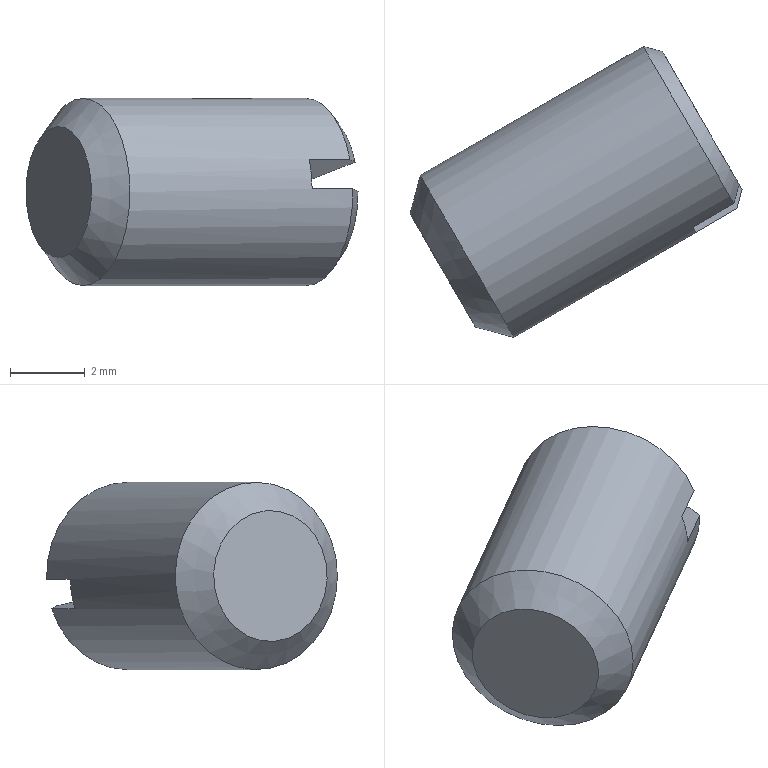Component | NX | GB-M5X8_2 | 1 solid | 10 faces | box 8.87 x 7.77 x 5 mm | volume 146 mm3 | plane 6 | cone 3 | cylinder 1 | commonest cylinder face diameters 5 x1
STEP:
#1=CARTESIAN_POINT('',(0.,0.,0.));
#2=DIRECTION('',(0.,0.,1.));
#3=DIRECTION('',(1.,0.,0.));
#4=AXIS2_PLACEMENT_3D('',#1,#2,#3);
#5=CARTESIAN_POINT('',(38.775,24.84,6.985));
#6=VERTEX_POINT('',#5);
#7=CARTESIAN_POINT('',(40.822,21.295,7.8));
#8=VERTEX_POINT('',#7);
#9=CARTESIAN_POINT('',(38.327,25.616,6.806));
#10=DIRECTION('',(0.4904,-0.8494,0.1953));
#11=VECTOR('',#10,1.);
#12=LINE('',#9,#11);
#13=CARTESIAN_POINT('',(39.837,23.,7.));
#14=DIRECTION('',(0.866,0.5,0.));
#15=DIRECTION('',(0.4904,-0.8494,0.1953));
#16=AXIS2_PLACEMENT_3D('',#13,#14,#15);
#17=PLANE('',#16);
#18=CARTESIAN_POINT('',(-3.,-0.4));
#19=DIRECTION('',(1.,0.));
#20=VECTOR('',#19,1.);
#21=LINE('',#18,#20);
#22=(GEOMETRIC_REPRESENTATION_CONTEXT(2)PARAMETRIC_REPRESENTATION_CONTEXT()REPRESENTATION_CONTEXT('',''));
#23=DEFINITIONAL_REPRESENTATION('',(#21),#22);
#24=PCURVE('',#17,#23);
#25=CARTESIAN_POINT('',(36.915,24.801,6.806));
#26=DIRECTION('',(-0.09764,0.1691,0.9807));
#27=DIRECTION('',(-0.866,-0.5,-0.));
#28=AXIS2_PLACEMENT_3D('',#25,#26,#27);
#29=PLANE('',#28);
#30=CARTESIAN_POINT('',(-1.63,0.));
#31=DIRECTION('',(0.,1.));
#32=VECTOR('',#31,1.);
#33=LINE('',#30,#32);
#34=(GEOMETRIC_REPRESENTATION_CONTEXT(2)PARAMETRIC_REPRESENTATION_CONTEXT()REPRESENTATION_CONTEXT('',''));
#35=DEFINITIONAL_REPRESENTATION('',(#33),#34);
#36=PCURVE('',#29,#35);
#37=SURFACE_CURVE('',#12,(#24,#36),.PCURVE_S1.);
#38=EDGE_CURVE('',#6,#8,#37,.T.);
#39=ORIENTED_EDGE('',*,*,#38,.F.);
#40=CARTESIAN_POINT('',(39.837,23.,7.));
#41=DIRECTION('',(0.866,0.5,-0.));
#42=DIRECTION('',(0.4904,-0.8494,0.1953));
#43=AXIS2_PLACEMENT_3D('',#40,#41,#42);
#44=CIRCLE('',#43,2.125);
#45=CARTESIAN_POINT('',(0.,0.));
#46=DIRECTION('',(1.,0.));
#47=AXIS2_PLACEMENT_2D('',#45,#46);
#48=CIRCLE('',#47,2.125);
#49=(GEOMETRIC_REPRESENTATION_CONTEXT(2)PARAMETRIC_REPRESENTATION_CONTEXT()REPRESENTATION_CONTEXT('',''));
#50=DEFINITIONAL_REPRESENTATION('',(#48),#49);
#51=PCURVE('',#17,#50);
#52=CARTESIAN_POINT('',(39.837,23.,7.));
#53=DIRECTION('',(-0.866,-0.5,0.));
#54=DIRECTION('',(-0.4904,0.8494,-0.1953));
#55=AXIS2_PLACEMENT_3D('',#52,#53,#54);
#56=CONICAL_SURFACE('',#55,2.125,0.7854);
#57=CARTESIAN_POINT('',(9.425,-0.));
#58=DIRECTION('',(-1.,0.));
#59=VECTOR('',#58,1.);
#60=LINE('',#57,#59);
#61=(GEOMETRIC_REPRESENTATION_CONTEXT(2)PARAMETRIC_REPRESENTATION_CONTEXT()REPRESENTATION_CONTEXT('',''));
#62=DEFINITIONAL_REPRESENTATION('',(#60),#61);
#63=PCURVE('',#56,#62);
#64=SURFACE_CURVE('',#44,(#51,#63),.PCURVE_S1.);
#65=EDGE_CURVE('',#6,#8,#64,.T.);
#66=ORIENTED_EDGE('',*,*,#65,.T.);
#67=EDGE_LOOP('',(#39,#66));
#68=FACE_BOUND('',#67,.T.);
#69=ADVANCED_FACE('',(#68),#17,.T.);
#70=CARTESIAN_POINT('',(38.263,24.976,6.91));
#71=VERTEX_POINT('',#70);
#72=CARTESIAN_POINT('',(38.263,24.976,6.91));
#73=CARTESIAN_POINT('',(38.434,24.931,6.935));
#74=CARTESIAN_POINT('',(38.604,24.886,6.96));
#75=CARTESIAN_POINT('',(38.775,24.84,6.985));
#76=B_SPLINE_CURVE_WITH_KNOTS('',3,(#72,#73,#74,#75),.UNSPECIFIED.,.F.,.F.,(4,4),(0.,1.),.PIECEWISE_BEZIER_KNOTS.);
#77=CARTESIAN_POINT('',(6.122,0.375));
#78=CARTESIAN_POINT('',(6.094,-0.));
#79=B_SPLINE_CURVE_WITH_KNOTS('',1,(#77,#78),.UNSPECIFIED.,.F.,.F.,(2,2),(0.,1.),.PIECEWISE_BEZIER_KNOTS.);
#80=(GEOMETRIC_REPRESENTATION_CONTEXT(2)PARAMETRIC_REPRESENTATION_CONTEXT()REPRESENTATION_CONTEXT('',''));
#81=DEFINITIONAL_REPRESENTATION('',(#79),#80);
#82=PCURVE('',#56,#81);
#83=CARTESIAN_POINT('',(-1.255,0.5322));
#84=CARTESIAN_POINT('',(-1.38,0.659));
#85=CARTESIAN_POINT('',(-1.505,0.7859));
#86=CARTESIAN_POINT('',(-1.63,0.913));
#87=B_SPLINE_CURVE_WITH_KNOTS('',3,(#83,#84,#85,#86),.UNSPECIFIED.,.F.,.F.,(4,4),(0.,1.),.PIECEWISE_BEZIER_KNOTS.);
#88=(GEOMETRIC_REPRESENTATION_CONTEXT(2)PARAMETRIC_REPRESENTATION_CONTEXT()REPRESENTATION_CONTEXT('',''));
#89=DEFINITIONAL_REPRESENTATION('',(#87),#88);
#90=PCURVE('',#29,#89);
#91=SURFACE_CURVE('',#76,(#82,#90),.PCURVE_S1.);
#92=EDGE_CURVE('',#71,#6,#91,.T.);
#93=ORIENTED_EDGE('',*,*,#92,.F.);
#94=CARTESIAN_POINT('',(40.683,20.784,7.874));
#95=VERTEX_POINT('',#94);
#96=CARTESIAN_POINT('',(39.512,22.812,7.));
#97=DIRECTION('',(-0.866,-0.5,0.));
#98=DIRECTION('',(0.4904,-0.8494,0.1953));
#99=AXIS2_PLACEMENT_3D('',#96,#97,#98);
#100=CIRCLE('',#99,2.5);
#101=CARTESIAN_POINT('',(3.142,0.375));
#102=DIRECTION('',(1.,-0.));
#103=VECTOR('',#102,1.);
#104=LINE('',#101,#103);
#105=(GEOMETRIC_REPRESENTATION_CONTEXT(2)PARAMETRIC_REPRESENTATION_CONTEXT()REPRESENTATION_CONTEXT('',''));
#106=DEFINITIONAL_REPRESENTATION('',(#104),#105);
#107=PCURVE('',#56,#106);
#108=CARTESIAN_POINT('',(39.837,23.,7.));
#109=DIRECTION('',(-0.866,-0.5,0.));
#110=DIRECTION('',(-0.4904,0.8494,-0.1953));
#111=AXIS2_PLACEMENT_3D('',#108,#109,#110);
#112=CYLINDRICAL_SURFACE('',#111,2.5);
#113=CARTESIAN_POINT('',(3.142,0.375));
#114=DIRECTION('',(1.,0.));
#115=VECTOR('',#114,1.);
#116=LINE('',#113,#115);
#117=(GEOMETRIC_REPRESENTATION_CONTEXT(2)PARAMETRIC_REPRESENTATION_CONTEXT()REPRESENTATION_CONTEXT('',''));
#118=DEFINITIONAL_REPRESENTATION('',(#116),#117);
#119=PCURVE('',#112,#118);
#120=SURFACE_CURVE('',#100,(#107,#119),.PCURVE_S1.);
#121=EDGE_CURVE('',#95,#71,#120,.T.);
#122=ORIENTED_EDGE('',*,*,#121,.F.);
#123=CARTESIAN_POINT('',(40.822,21.295,7.8));
#124=CARTESIAN_POINT('',(40.781,21.144,7.822));
#125=CARTESIAN_POINT('',(40.74,20.994,7.844));
#126=CARTESIAN_POINT('',(40.7,20.843,7.866));
#127=CARTESIAN_POINT('',(40.694,20.824,7.868));
#128=CARTESIAN_POINT('',(40.689,20.804,7.871));
#129=CARTESIAN_POINT('',(40.683,20.784,7.874));
#130=B_SPLINE_CURVE_WITH_KNOTS('',3,(#123,#124,#125,#126,#127,#128,#129),.UNSPECIFIED.,.F.,.F.,(4,3,4),(0.,0.8839,1.),.UNSPECIFIED.);
#131=CARTESIAN_POINT('',(3.331,-0.));
#132=CARTESIAN_POINT('',(3.302,0.375));
#133=B_SPLINE_CURVE_WITH_KNOTS('',1,(#131,#132),.UNSPECIFIED.,.F.,.F.,(2,2),(0.,1.),.PIECEWISE_BEZIER_KNOTS.);
#134=(GEOMETRIC_REPRESENTATION_CONTEXT(2)PARAMETRIC_REPRESENTATION_CONTEXT()REPRESENTATION_CONTEXT('',''));
#135=DEFINITIONAL_REPRESENTATION('',(#133),#134);
#136=PCURVE('',#56,#135);
#137=CARTESIAN_POINT('',(-1.63,5.087));
#138=CARTESIAN_POINT('',(-1.52,5.199));
#139=CARTESIAN_POINT('',(-1.409,5.312));
#140=CARTESIAN_POINT('',(-1.299,5.424));
#141=CARTESIAN_POINT('',(-1.284,5.438));
#142=CARTESIAN_POINT('',(-1.27,5.453));
#143=CARTESIAN_POINT('',(-1.255,5.468));
#144=B_SPLINE_CURVE_WITH_KNOTS('',3,(#137,#138,#139,#140,#141,#142,#143),.UNSPECIFIED.,.F.,.F.,(4,3,4),(0.,0.8839,1.),.UNSPECIFIED.);
#145=(GEOMETRIC_REPRESENTATION_CONTEXT(2)PARAMETRIC_REPRESENTATION_CONTEXT()REPRESENTATION_CONTEXT('',''));
#146=DEFINITIONAL_REPRESENTATION('',(#144),#145);
#147=PCURVE('',#29,#146);
#148=SURFACE_CURVE('',#130,(#136,#147),.PCURVE_S1.);
#149=EDGE_CURVE('',#8,#95,#148,.T.);
#150=ORIENTED_EDGE('',*,*,#149,.F.);
#151=ORIENTED_EDGE('',*,*,#65,.F.);
#152=EDGE_LOOP('',(#93,#122,#150,#151));
#153=FACE_BOUND('',#152,.T.);
#154=ADVANCED_FACE('',(#153),#56,.T.);
#155=ORIENTED_EDGE('',*,*,#121,.T.);
#156=CARTESIAN_POINT('',(37.176,24.349,6.91));
#157=VERTEX_POINT('',#156);
#158=CARTESIAN_POINT('',(38.588,25.164,6.91));
#159=DIRECTION('',(-0.866,-0.5,0.));
#160=VECTOR('',#159,1.);
#161=LINE('',#158,#160);
#162=CARTESIAN_POINT('',(6.122,-0.));
#163=DIRECTION('',(0.,1.));
#164=VECTOR('',#163,1.);
#165=LINE('',#162,#164);
#166=(GEOMETRIC_REPRESENTATION_CONTEXT(2)PARAMETRIC_REPRESENTATION_CONTEXT()REPRESENTATION_CONTEXT('',''));
#167=DEFINITIONAL_REPRESENTATION('',(#165),#166);
#168=PCURVE('',#112,#167);
#169=CARTESIAN_POINT('',(-1.63,0.5322));
#170=DIRECTION('',(1.,-0.));
#171=VECTOR('',#170,1.);
#172=LINE('',#169,#171);
#173=(GEOMETRIC_REPRESENTATION_CONTEXT(2)PARAMETRIC_REPRESENTATION_CONTEXT()REPRESENTATION_CONTEXT('',''));
#174=DEFINITIONAL_REPRESENTATION('',(#172),#173);
#175=PCURVE('',#29,#174);
#176=SURFACE_CURVE('',#161,(#168,#175),.PCURVE_S1.);
#177=EDGE_CURVE('',#71,#157,#176,.T.);
#178=ORIENTED_EDGE('',*,*,#177,.T.);
#179=CARTESIAN_POINT('',(37.254,24.213,6.126));
#180=VERTEX_POINT('',#179);
#181=CARTESIAN_POINT('',(38.426,22.185,7.));
#182=DIRECTION('',(0.866,0.5,0.));
#183=DIRECTION('',(0.4904,-0.8494,0.1953));
#184=AXIS2_PLACEMENT_3D('',#181,#182,#183);
#185=CIRCLE('',#184,2.5);
#186=CARTESIAN_POINT('',(9.425,1.63));
#187=DIRECTION('',(-1.,0.));
#188=VECTOR('',#187,1.);
#189=LINE('',#186,#188);
#190=(GEOMETRIC_REPRESENTATION_CONTEXT(2)PARAMETRIC_REPRESENTATION_CONTEXT()REPRESENTATION_CONTEXT('',''));
#191=DEFINITIONAL_REPRESENTATION('',(#189),#190);
#192=PCURVE('',#112,#191);
#193=CARTESIAN_POINT('',(38.426,22.185,7.));
#194=DIRECTION('',(0.866,0.5,0.));
#195=DIRECTION('',(0.4904,-0.8494,0.1953));
#196=AXIS2_PLACEMENT_3D('',#193,#194,#195);
#197=PLANE('',#196);
#198=CARTESIAN_POINT('',(0.,0.));
#199=DIRECTION('',(1.,-0.));
#200=AXIS2_PLACEMENT_2D('',#198,#199);
#201=CIRCLE('',#200,2.5);
#202=(GEOMETRIC_REPRESENTATION_CONTEXT(2)PARAMETRIC_REPRESENTATION_CONTEXT()REPRESENTATION_CONTEXT('',''));
#203=DEFINITIONAL_REPRESENTATION('',(#201),#202);
#204=PCURVE('',#197,#203);
#205=SURFACE_CURVE('',#185,(#192,#204),.PCURVE_S1.);
#206=EDGE_CURVE('',#180,#157,#205,.T.);
#207=ORIENTED_EDGE('',*,*,#206,.F.);
#208=CARTESIAN_POINT('',(32.387,21.403,6.126));
#209=VERTEX_POINT('',#208);
#210=CARTESIAN_POINT('',(37.254,24.213,6.126));
#211=CARTESIAN_POINT('',(32.387,21.403,6.126));
#212=B_SPLINE_CURVE_WITH_KNOTS('',1,(#210,#211),.UNSPECIFIED.,.F.,.F.,(2,2),(1.63,7.25),.PIECEWISE_BEZIER_KNOTS.);
#213=CARTESIAN_POINT('',(6.444,0.));
#214=DIRECTION('',(0.,1.));
#215=VECTOR('',#214,1.);
#216=LINE('',#213,#215);
#217=(GEOMETRIC_REPRESENTATION_CONTEXT(2)PARAMETRIC_REPRESENTATION_CONTEXT()REPRESENTATION_CONTEXT('',''));
#218=DEFINITIONAL_REPRESENTATION('',(#216),#217);
#219=PCURVE('',#112,#218);
#220=CARTESIAN_POINT('',(0.1607,0.));
#221=DIRECTION('',(0.,1.));
#222=VECTOR('',#221,1.);
#223=LINE('',#220,#222);
#224=(GEOMETRIC_REPRESENTATION_CONTEXT(2)PARAMETRIC_REPRESENTATION_CONTEXT()REPRESENTATION_CONTEXT('',''));
#225=DEFINITIONAL_REPRESENTATION('',(#223),#224);
#226=PCURVE('',#112,#225);
#227=SEAM_CURVE('',#212,(#219,#226),.PCURVE_S1.);
#228=EDGE_CURVE('',#180,#209,#227,.T.);
#229=ORIENTED_EDGE('',*,*,#228,.T.);
#230=CARTESIAN_POINT('',(34.784,17.252,7.488));
#231=VERTEX_POINT('',#230);
#232=CARTESIAN_POINT('',(33.558,19.375,7.));
#233=DIRECTION('',(0.866,0.5,0.));
#234=DIRECTION('',(0.4904,-0.8494,0.1953));
#235=AXIS2_PLACEMENT_3D('',#232,#233,#234);
#236=CIRCLE('',#235,2.5);
#237=CARTESIAN_POINT('',(9.425,7.25));
#238=DIRECTION('',(-1.,0.));
#239=VECTOR('',#238,1.);
#240=LINE('',#237,#239);
#241=(GEOMETRIC_REPRESENTATION_CONTEXT(2)PARAMETRIC_REPRESENTATION_CONTEXT()REPRESENTATION_CONTEXT('',''));
#242=DEFINITIONAL_REPRESENTATION('',(#240),#241);
#243=PCURVE('',#112,#242);
#244=CARTESIAN_POINT('',(33.558,19.375,7.));
#245=DIRECTION('',(0.866,0.5,0.));
#246=DIRECTION('',(0.4904,-0.8494,0.1953));
#247=AXIS2_PLACEMENT_3D('',#244,#245,#246);
#248=CONICAL_SURFACE('',#247,2.5,0.7854);
#249=CARTESIAN_POINT('',(0.,0.));
#250=DIRECTION('',(1.,-0.));
#251=VECTOR('',#250,1.);
#252=LINE('',#249,#251);
#253=(GEOMETRIC_REPRESENTATION_CONTEXT(2)PARAMETRIC_REPRESENTATION_CONTEXT()REPRESENTATION_CONTEXT('',''));
#254=DEFINITIONAL_REPRESENTATION('',(#252),#253);
#255=PCURVE('',#248,#254);
#256=SURFACE_CURVE('',#236,(#243,#255),.PCURVE_S1.);
#257=EDGE_CURVE('',#209,#231,#256,.T.);
#258=ORIENTED_EDGE('',*,*,#257,.T.);
#259=CARTESIAN_POINT('',(33.558,19.375,7.));
#260=DIRECTION('',(0.866,0.5,0.));
#261=DIRECTION('',(0.4904,-0.8494,0.1953));
#262=AXIS2_PLACEMENT_3D('',#259,#260,#261);
#263=CIRCLE('',#262,2.5);
#264=CARTESIAN_POINT('',(3.142,7.25));
#265=DIRECTION('',(-1.,0.));
#266=VECTOR('',#265,1.);
#267=LINE('',#264,#266);
#268=(GEOMETRIC_REPRESENTATION_CONTEXT(2)PARAMETRIC_REPRESENTATION_CONTEXT()REPRESENTATION_CONTEXT('',''));
#269=DEFINITIONAL_REPRESENTATION('',(#267),#268);
#270=PCURVE('',#112,#269);
#271=CARTESIAN_POINT('',(0.,-0.));
#272=DIRECTION('',(1.,0.));
#273=VECTOR('',#272,1.);
#274=LINE('',#271,#273);
#275=(GEOMETRIC_REPRESENTATION_CONTEXT(2)PARAMETRIC_REPRESENTATION_CONTEXT()REPRESENTATION_CONTEXT('',''));
#276=DEFINITIONAL_REPRESENTATION('',(#274),#275);
#277=PCURVE('',#248,#276);
#278=SURFACE_CURVE('',#263,(#270,#277),.PCURVE_S1.);
#279=EDGE_CURVE('',#231,#209,#278,.T.);
#280=ORIENTED_EDGE('',*,*,#279,.T.);
#281=ORIENTED_EDGE('',*,*,#228,.F.);
#282=CARTESIAN_POINT('',(38.341,24.841,6.126));
#283=VERTEX_POINT('',#282);
#284=CARTESIAN_POINT('',(38.666,25.028,6.126));
#285=DIRECTION('',(0.866,0.5,0.));
#286=VECTOR('',#285,1.);
#287=LINE('',#284,#286);
#288=CARTESIAN_POINT('',(0.1607,-0.));
#289=DIRECTION('',(0.,-1.));
#290=VECTOR('',#289,1.);
#291=LINE('',#288,#290);
#292=(GEOMETRIC_REPRESENTATION_CONTEXT(2)PARAMETRIC_REPRESENTATION_CONTEXT()REPRESENTATION_CONTEXT('',''));
#293=DEFINITIONAL_REPRESENTATION('',(#291),#292);
#294=PCURVE('',#112,#293);
#295=CARTESIAN_POINT('',(39.936,19.569,7.194));
#296=DIRECTION('',(0.09764,-0.1691,-0.9807));
#297=DIRECTION('',(0.866,0.5,0.));
#298=AXIS2_PLACEMENT_3D('',#295,#296,#297);
#299=PLANE('',#298);
#300=CARTESIAN_POINT('',(1.63,-5.468));
#301=DIRECTION('',(1.,0.));
#302=VECTOR('',#301,1.);
#303=LINE('',#300,#302);
#304=(GEOMETRIC_REPRESENTATION_CONTEXT(2)PARAMETRIC_REPRESENTATION_CONTEXT()REPRESENTATION_CONTEXT('',''));
#305=DEFINITIONAL_REPRESENTATION('',(#303),#304);
#306=PCURVE('',#299,#305);
#307=SURFACE_CURVE('',#287,(#294,#306),.PCURVE_S1.);
#308=EDGE_CURVE('',#180,#283,#307,.T.);
#309=ORIENTED_EDGE('',*,*,#308,.T.);
#310=CARTESIAN_POINT('',(40.762,20.649,7.09));
#311=VERTEX_POINT('',#310);
#312=CARTESIAN_POINT('',(39.512,22.812,7.));
#313=DIRECTION('',(-0.866,-0.5,0.));
#314=DIRECTION('',(0.4904,-0.8494,0.1953));
#315=AXIS2_PLACEMENT_3D('',#312,#313,#314);
#316=CIRCLE('',#315,2.5);
#317=CARTESIAN_POINT('',(-3.142,0.375));
#318=DIRECTION('',(1.,0.));
#319=VECTOR('',#318,1.);
#320=LINE('',#317,#319);
#321=(GEOMETRIC_REPRESENTATION_CONTEXT(2)PARAMETRIC_REPRESENTATION_CONTEXT()REPRESENTATION_CONTEXT('',''));
#322=DEFINITIONAL_REPRESENTATION('',(#320),#321);
#323=PCURVE('',#112,#322);
#324=CARTESIAN_POINT('',(39.837,23.,7.));
#325=DIRECTION('',(-0.866,-0.5,0.));
#326=DIRECTION('',(-0.4904,0.8494,-0.1953));
#327=AXIS2_PLACEMENT_3D('',#324,#325,#326);
#328=CONICAL_SURFACE('',#327,2.125,0.7854);
#329=CARTESIAN_POINT('',(-3.142,0.375));
#330=DIRECTION('',(1.,0.));
#331=VECTOR('',#330,1.);
#332=LINE('',#329,#331);
#333=(GEOMETRIC_REPRESENTATION_CONTEXT(2)PARAMETRIC_REPRESENTATION_CONTEXT()REPRESENTATION_CONTEXT('',''));
#334=DEFINITIONAL_REPRESENTATION('',(#332),#333);
#335=PCURVE('',#328,#334);
#336=SURFACE_CURVE('',#316,(#323,#335),.PCURVE_S1.);
#337=EDGE_CURVE('',#283,#311,#336,.T.);
#338=ORIENTED_EDGE('',*,*,#337,.T.);
#339=CARTESIAN_POINT('',(39.675,20.021,7.09));
#340=VERTEX_POINT('',#339);
#341=CARTESIAN_POINT('',(41.086,20.836,7.09));
#342=DIRECTION('',(-0.866,-0.5,0.));
#343=VECTOR('',#342,1.);
#344=LINE('',#341,#343);
#345=CARTESIAN_POINT('',(2.981,-0.));
#346=DIRECTION('',(0.,1.));
#347=VECTOR('',#346,1.);
#348=LINE('',#345,#347);
#349=(GEOMETRIC_REPRESENTATION_CONTEXT(2)PARAMETRIC_REPRESENTATION_CONTEXT()REPRESENTATION_CONTEXT('',''));
#350=DEFINITIONAL_REPRESENTATION('',(#348),#349);
#351=PCURVE('',#112,#350);
#352=CARTESIAN_POINT('',(1.63,-0.5322));
#353=DIRECTION('',(-1.,-0.));
#354=VECTOR('',#353,1.);
#355=LINE('',#352,#354);
#356=(GEOMETRIC_REPRESENTATION_CONTEXT(2)PARAMETRIC_REPRESENTATION_CONTEXT()REPRESENTATION_CONTEXT('',''));
#357=DEFINITIONAL_REPRESENTATION('',(#355),#356);
#358=PCURVE('',#299,#357);
#359=SURFACE_CURVE('',#344,(#351,#358),.PCURVE_S1.);
#360=EDGE_CURVE('',#311,#340,#359,.T.);
#361=ORIENTED_EDGE('',*,*,#360,.T.);
#362=CARTESIAN_POINT('',(39.597,20.157,7.874));
#363=VERTEX_POINT('',#362);
#364=CARTESIAN_POINT('',(38.426,22.185,7.));
#365=DIRECTION('',(0.866,0.5,0.));
#366=DIRECTION('',(0.4904,-0.8494,0.1953));
#367=AXIS2_PLACEMENT_3D('',#364,#365,#366);
#368=CIRCLE('',#367,2.5);
#369=CARTESIAN_POINT('',(9.425,1.63));
#370=DIRECTION('',(-1.,0.));
#371=VECTOR('',#370,1.);
#372=LINE('',#369,#371);
#373=(GEOMETRIC_REPRESENTATION_CONTEXT(2)PARAMETRIC_REPRESENTATION_CONTEXT()REPRESENTATION_CONTEXT('',''));
#374=DEFINITIONAL_REPRESENTATION('',(#372),#373);
#375=PCURVE('',#112,#374);
#376=CARTESIAN_POINT('',(0.,0.));
#377=DIRECTION('',(1.,-0.));
#378=AXIS2_PLACEMENT_2D('',#376,#377);
#379=CIRCLE('',#378,2.5);
#380=(GEOMETRIC_REPRESENTATION_CONTEXT(2)PARAMETRIC_REPRESENTATION_CONTEXT()REPRESENTATION_CONTEXT('',''));
#381=DEFINITIONAL_REPRESENTATION('',(#379),#380);
#382=PCURVE('',#197,#381);
#383=SURFACE_CURVE('',#368,(#375,#382),.PCURVE_S1.);
#384=EDGE_CURVE('',#363,#340,#383,.T.);
#385=ORIENTED_EDGE('',*,*,#384,.F.);
#386=CARTESIAN_POINT('',(41.008,20.972,7.874));
#387=DIRECTION('',(0.866,0.5,0.));
#388=VECTOR('',#387,1.);
#389=LINE('',#386,#388);
#390=CARTESIAN_POINT('',(3.302,-0.));
#391=DIRECTION('',(0.,-1.));
#392=VECTOR('',#391,1.);
#393=LINE('',#390,#392);
#394=(GEOMETRIC_REPRESENTATION_CONTEXT(2)PARAMETRIC_REPRESENTATION_CONTEXT()REPRESENTATION_CONTEXT('',''));
#395=DEFINITIONAL_REPRESENTATION('',(#393),#394);
#396=PCURVE('',#112,#395);
#397=CARTESIAN_POINT('',(-1.63,5.468));
#398=DIRECTION('',(-1.,0.));
#399=VECTOR('',#398,1.);
#400=LINE('',#397,#399);
#401=(GEOMETRIC_REPRESENTATION_CONTEXT(2)PARAMETRIC_REPRESENTATION_CONTEXT()REPRESENTATION_CONTEXT('',''));
#402=DEFINITIONAL_REPRESENTATION('',(#400),#401);
#403=PCURVE('',#29,#402);
#404=SURFACE_CURVE('',#389,(#396,#403),.PCURVE_S1.);
#405=EDGE_CURVE('',#363,#95,#404,.T.);
#406=ORIENTED_EDGE('',*,*,#405,.T.);
#407=EDGE_LOOP('',(#155,#178,#207,#229,#258,#280,#281,#309,#338,#361,#385,#406));
#408=FACE_BOUND('',#407,.T.);
#409=ADVANCED_FACE('',(#408),#112,.T.);
#410=CARTESIAN_POINT('',(40.9,21.16,7.015));
#411=VERTEX_POINT('',#410);
#412=CARTESIAN_POINT('',(38.853,24.705,6.2));
#413=VERTEX_POINT('',#412);
#414=CARTESIAN_POINT('',(41.347,20.384,7.194));
#415=DIRECTION('',(-0.4904,0.8494,-0.1953));
#416=VECTOR('',#415,1.);
#417=LINE('',#414,#416);
#418=CARTESIAN_POINT('',(39.837,23.,7.));
#419=DIRECTION('',(0.866,0.5,0.));
#420=DIRECTION('',(0.4904,-0.8494,0.1953));
#421=AXIS2_PLACEMENT_3D('',#418,#419,#420);
#422=PLANE('',#421);
#423=CARTESIAN_POINT('',(3.,0.4));
#424=DIRECTION('',(-1.,0.));
#425=VECTOR('',#424,1.);
#426=LINE('',#423,#425);
#427=(GEOMETRIC_REPRESENTATION_CONTEXT(2)PARAMETRIC_REPRESENTATION_CONTEXT()REPRESENTATION_CONTEXT('',''));
#428=DEFINITIONAL_REPRESENTATION('',(#426),#427);
#429=PCURVE('',#422,#428);
#430=CARTESIAN_POINT('',(1.63,-0.));
#431=DIRECTION('',(0.,-1.));
#432=VECTOR('',#431,1.);
#433=LINE('',#430,#432);
#434=(GEOMETRIC_REPRESENTATION_CONTEXT(2)PARAMETRIC_REPRESENTATION_CONTEXT()REPRESENTATION_CONTEXT('',''));
#435=DEFINITIONAL_REPRESENTATION('',(#433),#434);
#436=PCURVE('',#299,#435);
#437=SURFACE_CURVE('',#417,(#429,#436),.PCURVE_S1.);
#438=EDGE_CURVE('',#411,#413,#437,.T.);
#439=ORIENTED_EDGE('',*,*,#438,.F.);
#440=CARTESIAN_POINT('',(39.837,23.,7.));
#441=DIRECTION('',(0.866,0.5,-0.));
#442=DIRECTION('',(0.4904,-0.8494,0.1953));
#443=AXIS2_PLACEMENT_3D('',#440,#441,#442);
#444=CIRCLE('',#443,2.125);
#445=CARTESIAN_POINT('',(0.,0.));
#446=DIRECTION('',(1.,0.));
#447=AXIS2_PLACEMENT_2D('',#445,#446);
#448=CIRCLE('',#447,2.125);
#449=(GEOMETRIC_REPRESENTATION_CONTEXT(2)PARAMETRIC_REPRESENTATION_CONTEXT()REPRESENTATION_CONTEXT('',''));
#450=DEFINITIONAL_REPRESENTATION('',(#448),#449);
#451=PCURVE('',#422,#450);
#452=CARTESIAN_POINT('',(3.142,0.));
#453=DIRECTION('',(-1.,-0.));
#454=VECTOR('',#453,1.);
#455=LINE('',#452,#454);
#456=(GEOMETRIC_REPRESENTATION_CONTEXT(2)PARAMETRIC_REPRESENTATION_CONTEXT()REPRESENTATION_CONTEXT('',''));
#457=DEFINITIONAL_REPRESENTATION('',(#455),#456);
#458=PCURVE('',#328,#457);
#459=SURFACE_CURVE('',#444,(#451,#458),.PCURVE_S1.);
#460=EDGE_CURVE('',#411,#413,#459,.T.);
#461=ORIENTED_EDGE('',*,*,#460,.T.);
#462=EDGE_LOOP('',(#439,#461));
#463=FACE_BOUND('',#462,.T.);
#464=ADVANCED_FACE('',(#463),#422,.T.);
#465=CARTESIAN_POINT('',(33.767,17.514,7.342));
#466=VERTEX_POINT('',#465);
#467=CARTESIAN_POINT('',(32.909,19.,7.));
#468=DIRECTION('',(-0.866,-0.5,0.));
#469=DIRECTION('',(0.4904,-0.8494,0.1953));
#470=AXIS2_PLACEMENT_3D('',#467,#468,#469);
#471=CIRCLE('',#470,1.75);
#472=CARTESIAN_POINT('',(32.909,19.,7.));
#473=DIRECTION('',(0.866,0.5,0.));
#474=DIRECTION('',(0.4904,-0.8494,0.1953));
#475=AXIS2_PLACEMENT_3D('',#472,#473,#474);
#476=PLANE('',#475);
#477=CARTESIAN_POINT('',(1.75,0.));
#478=CARTESIAN_POINT('',(1.75,-3.031));
#479=CARTESIAN_POINT('',(-0.875,-1.516));
#480=CARTESIAN_POINT('',(-3.5,-0.));
#481=CARTESIAN_POINT('',(-0.875,1.516));
#482=CARTESIAN_POINT('',(1.75,3.031));
#483=CARTESIAN_POINT('',(1.75,0.));
#484=(BOUNDED_CURVE()B_SPLINE_CURVE(2,(#477,#478,#479,#480,#481,#482,#483),.UNSPECIFIED.,.T.,.F.)B_SPLINE_CURVE_WITH_KNOTS((1,2,2,2,2,1),(-2.094,0.,2.094,4.189,6.283,8.378),.UNSPECIFIED.)CURVE()GEOMETRIC_REPRESENTATION_ITEM()RATIONAL_B_SPLINE_CURVE((1.,0.5,1.,0.5,1.,0.5,1.))REPRESENTATION_ITEM(''));
#485=(GEOMETRIC_REPRESENTATION_CONTEXT(2)PARAMETRIC_REPRESENTATION_CONTEXT()REPRESENTATION_CONTEXT('',''));
#486=DEFINITIONAL_REPRESENTATION('',(#484),#485);
#487=PCURVE('',#476,#486);
#488=CARTESIAN_POINT('',(6.283,-0.75));
#489=DIRECTION('',(-1.,0.));
#490=VECTOR('',#489,1.);
#491=LINE('',#488,#490);
#492=(GEOMETRIC_REPRESENTATION_CONTEXT(2)PARAMETRIC_REPRESENTATION_CONTEXT()REPRESENTATION_CONTEXT('',''));
#493=DEFINITIONAL_REPRESENTATION('',(#491),#492);
#494=PCURVE('',#248,#493);
#495=SURFACE_CURVE('',#471,(#487,#494),.PCURVE_S1.);
#496=EDGE_CURVE('',#466,#466,#495,.T.);
#497=ORIENTED_EDGE('',*,*,#496,.T.);
#498=EDGE_LOOP('',(#497));
#499=FACE_BOUND('',#498,.T.);
#500=ADVANCED_FACE('',(#499),#476,.F.);
#501=CARTESIAN_POINT('',(40.762,20.649,7.09));
#502=CARTESIAN_POINT('',(40.808,20.819,7.065));
#503=CARTESIAN_POINT('',(40.854,20.989,7.04));
#504=CARTESIAN_POINT('',(40.9,21.16,7.015));
#505=B_SPLINE_CURVE_WITH_KNOTS('',3,(#501,#502,#503,#504),.UNSPECIFIED.,.F.,.F.,(4,4),(0.,1.),.PIECEWISE_BEZIER_KNOTS.);
#506=CARTESIAN_POINT('',(2.981,0.375));
#507=CARTESIAN_POINT('',(2.952,-0.));
#508=B_SPLINE_CURVE_WITH_KNOTS('',1,(#506,#507),.UNSPECIFIED.,.F.,.F.,(2,2),(0.,1.),.PIECEWISE_BEZIER_KNOTS.);
#509=(GEOMETRIC_REPRESENTATION_CONTEXT(2)PARAMETRIC_REPRESENTATION_CONTEXT()REPRESENTATION_CONTEXT('',''));
#510=DEFINITIONAL_REPRESENTATION('',(#508),#509);
#511=PCURVE('',#328,#510);
#512=CARTESIAN_POINT('',(1.255,-0.5322));
#513=CARTESIAN_POINT('',(1.38,-0.659));
#514=CARTESIAN_POINT('',(1.505,-0.7859));
#515=CARTESIAN_POINT('',(1.63,-0.913));
#516=B_SPLINE_CURVE_WITH_KNOTS('',3,(#512,#513,#514,#515),.UNSPECIFIED.,.F.,.F.,(4,4),(0.,1.),.PIECEWISE_BEZIER_KNOTS.);
#517=(GEOMETRIC_REPRESENTATION_CONTEXT(2)PARAMETRIC_REPRESENTATION_CONTEXT()REPRESENTATION_CONTEXT('',''));
#518=DEFINITIONAL_REPRESENTATION('',(#516),#517);
#519=PCURVE('',#299,#518);
#520=SURFACE_CURVE('',#505,(#511,#519),.PCURVE_S1.);
#521=EDGE_CURVE('',#311,#411,#520,.T.);
#522=ORIENTED_EDGE('',*,*,#521,.F.);
#523=ORIENTED_EDGE('',*,*,#337,.F.);
#524=CARTESIAN_POINT('',(38.853,24.705,6.2));
#525=CARTESIAN_POINT('',(38.702,24.745,6.178));
#526=CARTESIAN_POINT('',(38.551,24.785,6.156));
#527=CARTESIAN_POINT('',(38.401,24.825,6.134));
#528=CARTESIAN_POINT('',(38.381,24.83,6.132));
#529=CARTESIAN_POINT('',(38.361,24.836,6.129));
#530=CARTESIAN_POINT('',(38.341,24.841,6.126));
#531=B_SPLINE_CURVE_WITH_KNOTS('',3,(#524,#525,#526,#527,#528,#529,#530),.UNSPECIFIED.,.F.,.F.,(4,3,4),(0.,0.8839,1.),.UNSPECIFIED.);
#532=CARTESIAN_POINT('',(0.1894,-0.));
#533=CARTESIAN_POINT('',(0.1607,0.375));
#534=B_SPLINE_CURVE_WITH_KNOTS('',1,(#532,#533),.UNSPECIFIED.,.F.,.F.,(2,2),(0.,1.),.PIECEWISE_BEZIER_KNOTS.);
#535=(GEOMETRIC_REPRESENTATION_CONTEXT(2)PARAMETRIC_REPRESENTATION_CONTEXT()REPRESENTATION_CONTEXT('',''));
#536=DEFINITIONAL_REPRESENTATION('',(#534),#535);
#537=PCURVE('',#328,#536);
#538=CARTESIAN_POINT('',(1.63,-5.087));
#539=CARTESIAN_POINT('',(1.52,-5.199));
#540=CARTESIAN_POINT('',(1.409,-5.312));
#541=CARTESIAN_POINT('',(1.299,-5.424));
#542=CARTESIAN_POINT('',(1.284,-5.438));
#543=CARTESIAN_POINT('',(1.27,-5.453));
#544=CARTESIAN_POINT('',(1.255,-5.468));
#545=B_SPLINE_CURVE_WITH_KNOTS('',3,(#538,#539,#540,#541,#542,#543,#544),.UNSPECIFIED.,.F.,.F.,(4,3,4),(0.,0.8839,1.),.UNSPECIFIED.);
#546=(GEOMETRIC_REPRESENTATION_CONTEXT(2)PARAMETRIC_REPRESENTATION_CONTEXT()REPRESENTATION_CONTEXT('',''));
#547=DEFINITIONAL_REPRESENTATION('',(#545),#546);
#548=PCURVE('',#299,#547);
#549=SURFACE_CURVE('',#531,(#537,#548),.PCURVE_S1.);
#550=EDGE_CURVE('',#413,#283,#549,.T.);
#551=ORIENTED_EDGE('',*,*,#550,.F.);
#552=ORIENTED_EDGE('',*,*,#460,.F.);
#553=EDGE_LOOP('',(#522,#523,#551,#552));
#554=FACE_BOUND('',#553,.T.);
#555=ADVANCED_FACE('',(#554),#328,.T.);
#556=ORIENTED_EDGE('',*,*,#496,.F.);
#557=CARTESIAN_POINT('',(33.767,17.514,7.342));
#558=CARTESIAN_POINT('',(34.784,17.252,7.488));
#559=B_SPLINE_CURVE_WITH_KNOTS('',1,(#557,#558),.UNSPECIFIED.,.F.,.F.,(2,2),(-1.061,-0.),.PIECEWISE_BEZIER_KNOTS.);
#560=CARTESIAN_POINT('',(6.283,0.));
#561=DIRECTION('',(0.,1.));
#562=VECTOR('',#561,1.);
#563=LINE('',#560,#562);
#564=(GEOMETRIC_REPRESENTATION_CONTEXT(2)PARAMETRIC_REPRESENTATION_CONTEXT()REPRESENTATION_CONTEXT('',''));
#565=DEFINITIONAL_REPRESENTATION('',(#563),#564);
#566=PCURVE('',#248,#565);
#567=CARTESIAN_POINT('',(0.,0.));
#568=DIRECTION('',(0.,1.));
#569=VECTOR('',#568,1.);
#570=LINE('',#567,#569);
#571=(GEOMETRIC_REPRESENTATION_CONTEXT(2)PARAMETRIC_REPRESENTATION_CONTEXT()REPRESENTATION_CONTEXT('',''));
#572=DEFINITIONAL_REPRESENTATION('',(#570),#571);
#573=PCURVE('',#248,#572);
#574=SEAM_CURVE('',#559,(#566,#573),.PCURVE_S1.);
#575=EDGE_CURVE('',#466,#231,#574,.T.);
#576=ORIENTED_EDGE('',*,*,#575,.T.);
#577=ORIENTED_EDGE('',*,*,#257,.F.);
#578=ORIENTED_EDGE('',*,*,#279,.F.);
#579=ORIENTED_EDGE('',*,*,#575,.F.);
#580=EDGE_LOOP('',(#556,#576,#577,#578,#579));
#581=FACE_BOUND('',#580,.T.);
#582=ADVANCED_FACE('',(#581),#248,.T.);
#583=ORIENTED_EDGE('',*,*,#206,.T.);
#584=CARTESIAN_POINT('',(36.915,24.801,6.806));
#585=DIRECTION('',(-0.4904,0.8494,-0.1953));
#586=VECTOR('',#585,1.);
#587=LINE('',#584,#586);
#588=CARTESIAN_POINT('',(-3.,-0.4));
#589=DIRECTION('',(-1.,0.));
#590=VECTOR('',#589,1.);
#591=LINE('',#588,#590);
#592=(GEOMETRIC_REPRESENTATION_CONTEXT(2)PARAMETRIC_REPRESENTATION_CONTEXT()REPRESENTATION_CONTEXT('',''));
#593=DEFINITIONAL_REPRESENTATION('',(#591),#592);
#594=PCURVE('',#197,#593);
#595=CARTESIAN_POINT('',(0.,0.));
#596=DIRECTION('',(-0.,-1.));
#597=VECTOR('',#596,1.);
#598=LINE('',#595,#597);
#599=(GEOMETRIC_REPRESENTATION_CONTEXT(2)PARAMETRIC_REPRESENTATION_CONTEXT()REPRESENTATION_CONTEXT('',''));
#600=DEFINITIONAL_REPRESENTATION('',(#598),#599);
#601=PCURVE('',#29,#600);
#602=SURFACE_CURVE('',#587,(#594,#601),.PCURVE_S1.);
#603=EDGE_CURVE('',#363,#157,#602,.T.);
#604=ORIENTED_EDGE('',*,*,#603,.F.);
#605=ORIENTED_EDGE('',*,*,#384,.T.);
#606=CARTESIAN_POINT('',(39.936,19.569,7.194));
#607=DIRECTION('',(0.4904,-0.8494,0.1953));
#608=VECTOR('',#607,1.);
#609=LINE('',#606,#608);
#610=CARTESIAN_POINT('',(3.,0.4));
#611=DIRECTION('',(1.,0.));
#612=VECTOR('',#611,1.);
#613=LINE('',#610,#612);
#614=(GEOMETRIC_REPRESENTATION_CONTEXT(2)PARAMETRIC_REPRESENTATION_CONTEXT()REPRESENTATION_CONTEXT('',''));
#615=DEFINITIONAL_REPRESENTATION('',(#613),#614);
#616=PCURVE('',#197,#615);
#617=CARTESIAN_POINT('',(0.,0.));
#618=DIRECTION('',(-0.,1.));
#619=VECTOR('',#618,1.);
#620=LINE('',#617,#619);
#621=(GEOMETRIC_REPRESENTATION_CONTEXT(2)PARAMETRIC_REPRESENTATION_CONTEXT()REPRESENTATION_CONTEXT('',''));
#622=DEFINITIONAL_REPRESENTATION('',(#620),#621);
#623=PCURVE('',#299,#622);
#624=SURFACE_CURVE('',#609,(#616,#623),.PCURVE_S1.);
#625=EDGE_CURVE('',#180,#340,#624,.T.);
#626=ORIENTED_EDGE('',*,*,#625,.F.);
#627=EDGE_LOOP('',(#583,#604,#605,#626));
#628=FACE_BOUND('',#627,.T.);
#629=ADVANCED_FACE('',(#628),#197,.T.);
#630=ORIENTED_EDGE('',*,*,#92,.T.);
#631=ORIENTED_EDGE('',*,*,#38,.T.);
#632=ORIENTED_EDGE('',*,*,#149,.T.);
#633=ORIENTED_EDGE('',*,*,#405,.F.);
#634=ORIENTED_EDGE('',*,*,#603,.T.);
#635=ORIENTED_EDGE('',*,*,#177,.F.);
#636=EDGE_LOOP('',(#630,#631,#632,#633,#634,#635));
#637=FACE_BOUND('',#636,.T.);
#638=ADVANCED_FACE('',(#637),#29,.F.);
#639=ORIENTED_EDGE('',*,*,#521,.T.);
#640=ORIENTED_EDGE('',*,*,#438,.T.);
#641=ORIENTED_EDGE('',*,*,#550,.T.);
#642=ORIENTED_EDGE('',*,*,#308,.F.);
#643=ORIENTED_EDGE('',*,*,#625,.T.);
#644=ORIENTED_EDGE('',*,*,#360,.F.);
#645=EDGE_LOOP('',(#639,#640,#641,#642,#643,#644));
#646=FACE_BOUND('',#645,.T.);
#647=ADVANCED_FACE('',(#646),#299,.F.);
#648=CLOSED_SHELL('',(#69,#154,#409,#464,#500,#555,#582,#629,#638,#647));
#649=MANIFOLD_SOLID_BREP('',#648);
#650=(LENGTH_UNIT()NAMED_UNIT(*)SI_UNIT(.MILLI.,.METRE.));
#651=UNCERTAINTY_MEASURE_WITH_UNIT(LENGTH_MEASURE(0.001),#650,'','');
#652=(NAMED_UNIT(*)PLANE_ANGLE_UNIT()SI_UNIT($,.RADIAN.));
#653=(NAMED_UNIT(*)SI_UNIT($,.STERADIAN.)SOLID_ANGLE_UNIT());
#654=(GEOMETRIC_REPRESENTATION_CONTEXT(3)GLOBAL_UNCERTAINTY_ASSIGNED_CONTEXT((#651))GLOBAL_UNIT_ASSIGNED_CONTEXT((#650,#652,#653))REPRESENTATION_CONTEXT('',''));
#655=ADVANCED_BREP_SHAPE_REPRESENTATION('',(#4,#649),#654);